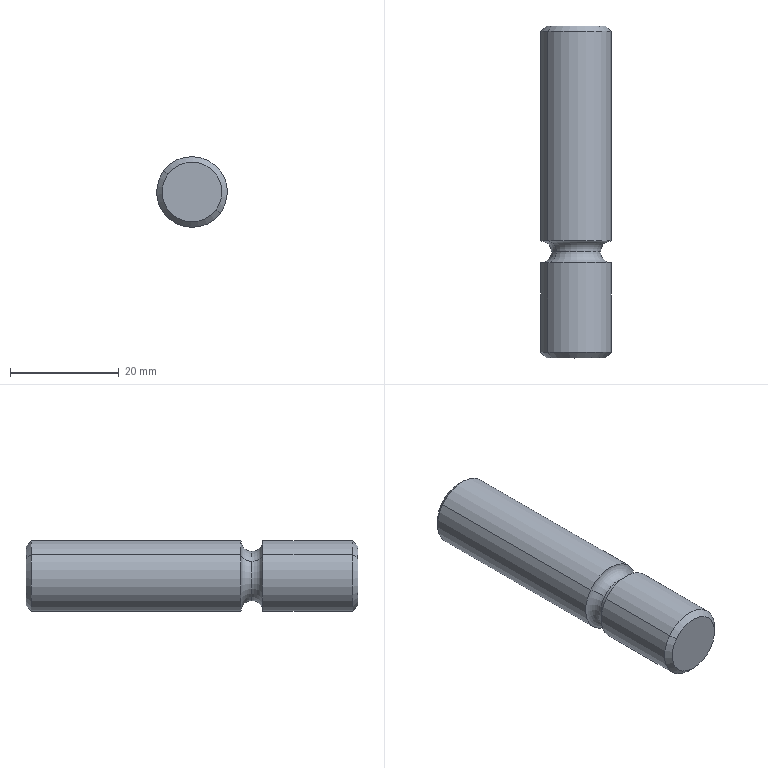Component | SolidWorks | 18-1 | 1 solid | 14 faces | box 13 x 61 x 13 mm | volume 7835 mm3 | torus 4 | cylinder 4 | cone 4 | plane 2 | commonest cylinder face diameters 13 x4
build123d program:
from build123d import *

# Parameters (mm, degrees)
SKETCH1_R           = 6.5
BOSS_EXTRUDE1_DEPTH = 61
CHAMFER1_SIZE       = 1
SKETCH2_R           = 2


with BuildPart() as part:
    # Sketch1 → Boss-Extrude1 (new body)
    with BuildSketch(Plane(origin=(0, 0, 0), x_dir=(0, 0, -1), z_dir=(1, 0, 0))):
        with Locations(Location((0, 0, 0), (0, 0, 180))):
            Circle(SKETCH1_R)
    extrude(amount=BOSS_EXTRUDE1_DEPTH)

    # Chamfer1
    chamfer1_edges = [part.edges().sort_by_distance(p)[0] for p in [
        (0, 0, -6.5),
        (61, 0, -6.5),
    ]]
    chamfer(chamfer1_edges, length=CHAMFER1_SIZE)

    # Sketch2 → Cut-Revolve1 (revolve, cut)
    with BuildSketch(Plane.XY, mode=Mode.PRIVATE) as cut_revolve1_sk:
        with Locations((19.5, 6.5)):
            Circle(SKETCH2_R)
    revolve(cut_revolve1_sk.sketch.rotate(Axis((0, 0, 0), (1, 0, 0)), 90), axis=Axis((0, 0, 0), (1, 0, 0)), mode=Mode.SUBTRACT)


solid = part.part

# Placed as in the assembly
solid = solid.moved(Location((-149.043, 247.491, 673.144), (0, 0, 90)))
STEP:
#1=COLOUR_RGB('',0.7922,0.8196,0.9333);
#2=FILL_AREA_STYLE_COLOUR('',#1);
#3=FILL_AREA_STYLE('',(#2));
#4=SURFACE_STYLE_FILL_AREA(#3);
#5=SURFACE_SIDE_STYLE('',(#4));
#6=SURFACE_STYLE_USAGE(.BOTH.,#5);
#7=PRESENTATION_STYLE_ASSIGNMENT((#6));
#8=CARTESIAN_POINT('',(-6.072,10.433,26.656));
#9=VERTEX_POINT('',#8);
#10=CARTESIAN_POINT('',(-6.009,10.511,26.609));
#11=VERTEX_POINT('',#10);
#12=CARTESIAN_POINT('',(-6.072,10.511,26.656));
#13=DIRECTION('',(0.6039,0.,0.797));
#14=DIRECTION('',(0.797,0.,-0.6039));
#15=AXIS2_PLACEMENT_3D('',#12,#13,#14);
#16=CIRCLE('',#15,0.07874);
#17=EDGE_CURVE('',#9,#11,#16,.T.);
#18=ORIENTED_EDGE('',*,*,#17,.T.);
#19=CARTESIAN_POINT('',(-5.727,10.511,26.395));
#20=VERTEX_POINT('',#19);
#21=CARTESIAN_POINT('',(-5.868,10.511,26.502));
#22=DIRECTION('',(0.,-1.,0.));
#23=DIRECTION('',(0.,0.,-1.));
#24=AXIS2_PLACEMENT_3D('',#21,#22,#23);
#25=CIRCLE('',#24,0.1772);
#26=EDGE_CURVE('',#11,#20,#25,.T.);
#27=ORIENTED_EDGE('',*,*,#26,.T.);
#28=CARTESIAN_POINT('',(-5.664,10.433,26.347));
#29=VERTEX_POINT('',#28);
#30=CARTESIAN_POINT('',(-5.664,10.511,26.347));
#31=DIRECTION('',(-0.6039,-0.,-0.797));
#32=DIRECTION('',(-0.797,0.,0.6039));
#33=AXIS2_PLACEMENT_3D('',#30,#31,#32);
#34=CIRCLE('',#33,0.07874);
#35=EDGE_CURVE('',#29,#20,#34,.T.);
#36=ORIENTED_EDGE('',*,*,#35,.F.);
#37=CARTESIAN_POINT('',(-5.868,10.433,26.502));
#38=DIRECTION('',(-0.,1.,-0.));
#39=DIRECTION('',(0.797,0.,-0.6039));
#40=AXIS2_PLACEMENT_3D('',#37,#38,#39);
#41=CIRCLE('',#40,0.2559);
#42=EDGE_CURVE('',#29,#9,#41,.T.);
#43=ORIENTED_EDGE('',*,*,#42,.T.);
#44=EDGE_LOOP('',(#18,#27,#36,#43));
#45=FACE_OUTER_BOUND('',#44,.T.);
#46=CARTESIAN_POINT('',(-5.868,10.511,26.502));
#47=DIRECTION('',(0.,-1.,0.));
#48=DIRECTION('',(-0.797,0.,0.6039));
#49=AXIS2_PLACEMENT_3D('',#46,#47,#48);
#50=TOROIDAL_SURFACE('',#49,0.2559,0.07874);
#51=ADVANCED_FACE('',(#45),#50,.F.);
#52=ORIENTED_EDGE('',*,*,#35,.T.);
#53=CARTESIAN_POINT('',(-5.868,10.511,26.502));
#54=DIRECTION('',(0.,-1.,0.));
#55=DIRECTION('',(0.,0.,-1.));
#56=AXIS2_PLACEMENT_3D('',#53,#54,#55);
#57=CIRCLE('',#56,0.1772);
#58=EDGE_CURVE('',#20,#11,#57,.T.);
#59=ORIENTED_EDGE('',*,*,#58,.T.);
#60=ORIENTED_EDGE('',*,*,#17,.F.);
#61=CARTESIAN_POINT('',(-5.868,10.433,26.502));
#62=DIRECTION('',(-0.,1.,-0.));
#63=DIRECTION('',(0.797,0.,-0.6039));
#64=AXIS2_PLACEMENT_3D('',#61,#62,#63);
#65=CIRCLE('',#64,0.2559);
#66=EDGE_CURVE('',#9,#29,#65,.T.);
#67=ORIENTED_EDGE('',*,*,#66,.T.);
#68=EDGE_LOOP('',(#52,#59,#60,#67));
#69=FACE_OUTER_BOUND('',#68,.T.);
#70=CARTESIAN_POINT('',(-5.868,10.511,26.502));
#71=DIRECTION('',(0.,-1.,0.));
#72=DIRECTION('',(-0.797,0.,0.6039));
#73=AXIS2_PLACEMENT_3D('',#70,#71,#72);
#74=TOROIDAL_SURFACE('',#73,0.2559,0.07874);
#75=ADVANCED_FACE('',(#69),#74,.F.);
#76=CARTESIAN_POINT('',(-6.072,12.106,26.656));
#77=VERTEX_POINT('',#76);
#78=CARTESIAN_POINT('',(-5.664,12.106,26.347));
#79=VERTEX_POINT('',#78);
#80=CARTESIAN_POINT('',(-5.868,12.106,26.502));
#81=DIRECTION('',(0.,-1.,0.));
#82=DIRECTION('',(0.797,0.,-0.6039));
#83=AXIS2_PLACEMENT_3D('',#80,#81,#82);
#84=CIRCLE('',#83,0.2559);
#85=EDGE_CURVE('',#77,#79,#84,.T.);
#86=ORIENTED_EDGE('',*,*,#85,.T.);
#87=CARTESIAN_POINT('',(-5.664,10.59,26.347));
#88=VERTEX_POINT('',#87);
#89=CARTESIAN_POINT('',(-5.664,12.145,26.347));
#90=DIRECTION('',(0.,-1.,0.));
#91=VECTOR('',#90,39.37);
#92=LINE('',#89,#91);
#93=EDGE_CURVE('',#79,#88,#92,.T.);
#94=ORIENTED_EDGE('',*,*,#93,.T.);
#95=CARTESIAN_POINT('',(-6.072,10.59,26.656));
#96=VERTEX_POINT('',#95);
#97=CARTESIAN_POINT('',(-5.868,10.59,26.502));
#98=DIRECTION('',(0.,-1.,0.));
#99=DIRECTION('',(-0.797,0.,0.6039));
#100=AXIS2_PLACEMENT_3D('',#97,#98,#99);
#101=CIRCLE('',#100,0.2559);
#102=EDGE_CURVE('',#96,#88,#101,.T.);
#103=ORIENTED_EDGE('',*,*,#102,.F.);
#104=CARTESIAN_POINT('',(-6.072,12.145,26.656));
#105=DIRECTION('',(0.,-1.,0.));
#106=VECTOR('',#105,39.37);
#107=LINE('',#104,#106);
#108=EDGE_CURVE('',#77,#96,#107,.T.);
#109=ORIENTED_EDGE('',*,*,#108,.F.);
#110=EDGE_LOOP('',(#86,#94,#103,#109));
#111=FACE_OUTER_BOUND('',#110,.T.);
#112=CARTESIAN_POINT('',(-5.868,12.145,26.502));
#113=DIRECTION('',(0.,-1.,0.));
#114=DIRECTION('',(-0.797,0.,0.6039));
#115=AXIS2_PLACEMENT_3D('',#112,#113,#114);
#116=CYLINDRICAL_SURFACE('',#115,0.2559);
#117=ADVANCED_FACE('',(#111),#116,.T.);
#118=CARTESIAN_POINT('',(-5.695,12.145,26.371));
#119=VERTEX_POINT('',#118);
#120=CARTESIAN_POINT('',(-6.04,12.145,26.632));
#121=VERTEX_POINT('',#120);
#122=CARTESIAN_POINT('',(-5.868,12.145,26.502));
#123=DIRECTION('',(-0.,1.,-0.));
#124=DIRECTION('',(0.797,0.,-0.6039));
#125=AXIS2_PLACEMENT_3D('',#122,#123,#124);
#126=CIRCLE('',#125,0.2165);
#127=EDGE_CURVE('',#119,#121,#126,.T.);
#128=ORIENTED_EDGE('',*,*,#127,.F.);
#129=CARTESIAN_POINT('',(-5.695,12.145,26.371));
#130=DIRECTION('',(0.5636,-0.7071,-0.427));
#131=VECTOR('',#130,39.37);
#132=LINE('',#129,#131);
#133=EDGE_CURVE('',#119,#79,#132,.T.);
#134=ORIENTED_EDGE('',*,*,#133,.T.);
#135=ORIENTED_EDGE('',*,*,#85,.F.);
#136=CARTESIAN_POINT('',(-6.04,12.145,26.632));
#137=DIRECTION('',(-0.5636,-0.7071,0.427));
#138=VECTOR('',#137,39.37);
#139=LINE('',#136,#138);
#140=EDGE_CURVE('',#121,#77,#139,.T.);
#141=ORIENTED_EDGE('',*,*,#140,.F.);
#142=EDGE_LOOP('',(#128,#134,#135,#141));
#143=FACE_OUTER_BOUND('',#142,.T.);
#144=CARTESIAN_POINT('',(-5.868,12.145,26.502));
#145=DIRECTION('',(0.,-1.,0.));
#146=DIRECTION('',(-0.797,0.,0.6039));
#147=AXIS2_PLACEMENT_3D('',#144,#145,#146);
#148=CONICAL_SURFACE('',#147,0.2165,0.7854);
#149=ADVANCED_FACE('',(#143),#148,.T.);
#150=ORIENTED_EDGE('',*,*,#58,.F.);
#151=CARTESIAN_POINT('',(-5.664,10.511,26.347));
#152=DIRECTION('',(-0.6039,-0.,-0.797));
#153=DIRECTION('',(-0.797,0.,0.6039));
#154=AXIS2_PLACEMENT_3D('',#151,#152,#153);
#155=CIRCLE('',#154,0.07874);
#156=EDGE_CURVE('',#20,#88,#155,.T.);
#157=ORIENTED_EDGE('',*,*,#156,.T.);
#158=CARTESIAN_POINT('',(-5.868,10.59,26.502));
#159=DIRECTION('',(0.,-1.,0.));
#160=DIRECTION('',(-0.797,0.,0.6039));
#161=AXIS2_PLACEMENT_3D('',#158,#159,#160);
#162=CIRCLE('',#161,0.2559);
#163=EDGE_CURVE('',#88,#96,#162,.T.);
#164=ORIENTED_EDGE('',*,*,#163,.T.);
#165=CARTESIAN_POINT('',(-6.072,10.511,26.656));
#166=DIRECTION('',(0.6039,0.,0.797));
#167=DIRECTION('',(0.797,0.,-0.6039));
#168=AXIS2_PLACEMENT_3D('',#165,#166,#167);
#169=CIRCLE('',#168,0.07874);
#170=EDGE_CURVE('',#11,#96,#169,.T.);
#171=ORIENTED_EDGE('',*,*,#170,.F.);
#172=EDGE_LOOP('',(#150,#157,#164,#171));
#173=FACE_OUTER_BOUND('',#172,.T.);
#174=CARTESIAN_POINT('',(-5.868,10.511,26.502));
#175=DIRECTION('',(0.,-1.,0.));
#176=DIRECTION('',(-0.797,0.,0.6039));
#177=AXIS2_PLACEMENT_3D('',#174,#175,#176);
#178=TOROIDAL_SURFACE('',#177,0.2559,0.07874);
#179=ADVANCED_FACE('',(#173),#178,.F.);
#180=CARTESIAN_POINT('',(-6.04,9.744,26.632));
#181=VERTEX_POINT('',#180);
#182=CARTESIAN_POINT('',(-5.695,9.744,26.371));
#183=VERTEX_POINT('',#182);
#184=CARTESIAN_POINT('',(-5.868,9.744,26.502));
#185=DIRECTION('',(0.,-1.,0.));
#186=DIRECTION('',(0.797,0.,-0.6039));
#187=AXIS2_PLACEMENT_3D('',#184,#185,#186);
#188=CIRCLE('',#187,0.2165);
#189=EDGE_CURVE('',#181,#183,#188,.T.);
#190=ORIENTED_EDGE('',*,*,#189,.F.);
#191=CARTESIAN_POINT('',(-6.072,9.783,26.656));
#192=VERTEX_POINT('',#191);
#193=CARTESIAN_POINT('',(-6.072,9.783,26.656));
#194=DIRECTION('',(-0.5636,0.7071,0.427));
#195=VECTOR('',#194,39.37);
#196=LINE('',#193,#195);
#197=EDGE_CURVE('',#181,#192,#196,.T.);
#198=ORIENTED_EDGE('',*,*,#197,.T.);
#199=CARTESIAN_POINT('',(-5.664,9.783,26.347));
#200=VERTEX_POINT('',#199);
#201=CARTESIAN_POINT('',(-5.868,9.783,26.502));
#202=DIRECTION('',(-0.,1.,-0.));
#203=DIRECTION('',(0.797,0.,-0.6039));
#204=AXIS2_PLACEMENT_3D('',#201,#202,#203);
#205=CIRCLE('',#204,0.2559);
#206=EDGE_CURVE('',#200,#192,#205,.T.);
#207=ORIENTED_EDGE('',*,*,#206,.F.);
#208=CARTESIAN_POINT('',(-5.664,9.783,26.347));
#209=DIRECTION('',(0.5636,0.7071,-0.427));
#210=VECTOR('',#209,39.37);
#211=LINE('',#208,#210);
#212=EDGE_CURVE('',#183,#200,#211,.T.);
#213=ORIENTED_EDGE('',*,*,#212,.F.);
#214=EDGE_LOOP('',(#190,#198,#207,#213));
#215=FACE_OUTER_BOUND('',#214,.T.);
#216=CARTESIAN_POINT('',(-5.868,9.783,26.502));
#217=DIRECTION('',(-0.,1.,-0.));
#218=DIRECTION('',(0.797,0.,-0.6039));
#219=AXIS2_PLACEMENT_3D('',#216,#217,#218);
#220=CONICAL_SURFACE('',#219,0.2559,0.7854);
#221=ADVANCED_FACE('',(#215),#220,.T.);
#222=ORIENTED_EDGE('',*,*,#42,.F.);
#223=CARTESIAN_POINT('',(-5.664,12.145,26.347));
#224=DIRECTION('',(0.,-1.,0.));
#225=VECTOR('',#224,39.37);
#226=LINE('',#223,#225);
#227=EDGE_CURVE('',#29,#200,#226,.T.);
#228=ORIENTED_EDGE('',*,*,#227,.T.);
#229=ORIENTED_EDGE('',*,*,#206,.T.);
#230=CARTESIAN_POINT('',(-6.072,12.145,26.656));
#231=DIRECTION('',(0.,-1.,0.));
#232=VECTOR('',#231,39.37);
#233=LINE('',#230,#232);
#234=EDGE_CURVE('',#9,#192,#233,.T.);
#235=ORIENTED_EDGE('',*,*,#234,.F.);
#236=EDGE_LOOP('',(#222,#228,#229,#235));
#237=FACE_OUTER_BOUND('',#236,.T.);
#238=CARTESIAN_POINT('',(-5.868,12.145,26.502));
#239=DIRECTION('',(0.,-1.,0.));
#240=DIRECTION('',(-0.797,0.,0.6039));
#241=AXIS2_PLACEMENT_3D('',#238,#239,#240);
#242=CYLINDRICAL_SURFACE('',#241,0.2559);
#243=ADVANCED_FACE('',(#237),#242,.T.);
#244=ORIENTED_EDGE('',*,*,#227,.F.);
#245=ORIENTED_EDGE('',*,*,#66,.F.);
#246=ORIENTED_EDGE('',*,*,#234,.T.);
#247=CARTESIAN_POINT('',(-5.868,9.783,26.502));
#248=DIRECTION('',(-0.,1.,-0.));
#249=DIRECTION('',(0.797,0.,-0.6039));
#250=AXIS2_PLACEMENT_3D('',#247,#248,#249);
#251=CIRCLE('',#250,0.2559);
#252=EDGE_CURVE('',#192,#200,#251,.T.);
#253=ORIENTED_EDGE('',*,*,#252,.T.);
#254=EDGE_LOOP('',(#244,#245,#246,#253));
#255=FACE_OUTER_BOUND('',#254,.T.);
#256=CARTESIAN_POINT('',(-5.868,12.145,26.502));
#257=DIRECTION('',(0.,-1.,0.));
#258=DIRECTION('',(-0.797,0.,0.6039));
#259=AXIS2_PLACEMENT_3D('',#256,#257,#258);
#260=CYLINDRICAL_SURFACE('',#259,0.2559);
#261=ADVANCED_FACE('',(#255),#260,.T.);
#262=CARTESIAN_POINT('',(-5.868,9.744,26.502));
#263=DIRECTION('',(0.,-1.,0.));
#264=DIRECTION('',(0.797,0.,-0.6039));
#265=AXIS2_PLACEMENT_3D('',#262,#263,#264);
#266=CIRCLE('',#265,0.2165);
#267=EDGE_CURVE('',#183,#181,#266,.T.);
#268=ORIENTED_EDGE('',*,*,#267,.T.);
#269=ORIENTED_EDGE('',*,*,#189,.T.);
#270=EDGE_LOOP('',(#268,#269));
#271=FACE_OUTER_BOUND('',#270,.T.);
#272=CARTESIAN_POINT('',(-5.868,9.744,26.502));
#273=DIRECTION('',(-0.,1.,-0.));
#274=DIRECTION('',(0.797,-0.,-0.6039));
#275=AXIS2_PLACEMENT_3D('',#272,#273,#274);
#276=PLANE('',#275);
#277=ADVANCED_FACE('',(#271),#276,.F.);
#278=ORIENTED_EDGE('',*,*,#197,.F.);
#279=ORIENTED_EDGE('',*,*,#267,.F.);
#280=ORIENTED_EDGE('',*,*,#212,.T.);
#281=ORIENTED_EDGE('',*,*,#252,.F.);
#282=EDGE_LOOP('',(#278,#279,#280,#281));
#283=FACE_OUTER_BOUND('',#282,.T.);
#284=CARTESIAN_POINT('',(-5.868,9.783,26.502));
#285=DIRECTION('',(-0.,1.,-0.));
#286=DIRECTION('',(0.797,0.,-0.6039));
#287=AXIS2_PLACEMENT_3D('',#284,#285,#286);
#288=CONICAL_SURFACE('',#287,0.2559,0.7854);
#289=ADVANCED_FACE('',(#283),#288,.T.);
#290=ORIENTED_EDGE('',*,*,#26,.F.);
#291=ORIENTED_EDGE('',*,*,#170,.T.);
#292=ORIENTED_EDGE('',*,*,#102,.T.);
#293=ORIENTED_EDGE('',*,*,#156,.F.);
#294=EDGE_LOOP('',(#290,#291,#292,#293));
#295=FACE_OUTER_BOUND('',#294,.T.);
#296=CARTESIAN_POINT('',(-5.868,10.511,26.502));
#297=DIRECTION('',(0.,-1.,0.));
#298=DIRECTION('',(-0.797,0.,0.6039));
#299=AXIS2_PLACEMENT_3D('',#296,#297,#298);
#300=TOROIDAL_SURFACE('',#299,0.2559,0.07874);
#301=ADVANCED_FACE('',(#295),#300,.F.);
#302=CARTESIAN_POINT('',(-5.868,12.145,26.502));
#303=DIRECTION('',(-0.,1.,-0.));
#304=DIRECTION('',(0.797,0.,-0.6039));
#305=AXIS2_PLACEMENT_3D('',#302,#303,#304);
#306=CIRCLE('',#305,0.2165);
#307=EDGE_CURVE('',#121,#119,#306,.T.);
#308=ORIENTED_EDGE('',*,*,#307,.T.);
#309=ORIENTED_EDGE('',*,*,#127,.T.);
#310=EDGE_LOOP('',(#308,#309));
#311=FACE_OUTER_BOUND('',#310,.T.);
#312=CARTESIAN_POINT('',(-5.868,12.145,26.502));
#313=DIRECTION('',(-0.,1.,-0.));
#314=DIRECTION('',(0.797,-0.,-0.6039));
#315=AXIS2_PLACEMENT_3D('',#312,#313,#314);
#316=PLANE('',#315);
#317=ADVANCED_FACE('',(#311),#316,.T.);
#318=ORIENTED_EDGE('',*,*,#133,.F.);
#319=ORIENTED_EDGE('',*,*,#307,.F.);
#320=ORIENTED_EDGE('',*,*,#140,.T.);
#321=CARTESIAN_POINT('',(-5.868,12.106,26.502));
#322=DIRECTION('',(0.,-1.,0.));
#323=DIRECTION('',(0.797,0.,-0.6039));
#324=AXIS2_PLACEMENT_3D('',#321,#322,#323);
#325=CIRCLE('',#324,0.2559);
#326=EDGE_CURVE('',#79,#77,#325,.T.);
#327=ORIENTED_EDGE('',*,*,#326,.F.);
#328=EDGE_LOOP('',(#318,#319,#320,#327));
#329=FACE_OUTER_BOUND('',#328,.T.);
#330=CARTESIAN_POINT('',(-5.868,12.145,26.502));
#331=DIRECTION('',(0.,-1.,0.));
#332=DIRECTION('',(-0.797,0.,0.6039));
#333=AXIS2_PLACEMENT_3D('',#330,#331,#332);
#334=CONICAL_SURFACE('',#333,0.2165,0.7854);
#335=ADVANCED_FACE('',(#329),#334,.T.);
#336=ORIENTED_EDGE('',*,*,#93,.F.);
#337=ORIENTED_EDGE('',*,*,#326,.T.);
#338=ORIENTED_EDGE('',*,*,#108,.T.);
#339=ORIENTED_EDGE('',*,*,#163,.F.);
#340=EDGE_LOOP('',(#336,#337,#338,#339));
#341=FACE_OUTER_BOUND('',#340,.T.);
#342=CARTESIAN_POINT('',(-5.868,12.145,26.502));
#343=DIRECTION('',(0.,-1.,0.));
#344=DIRECTION('',(-0.797,0.,0.6039));
#345=AXIS2_PLACEMENT_3D('',#342,#343,#344);
#346=CYLINDRICAL_SURFACE('',#345,0.2559);
#347=ADVANCED_FACE('',(#341),#346,.T.);
#348=CLOSED_SHELL('',(#51,#75,#117,#149,#179,#221,#243,#261,#277,#289,#301,#317,#335,#347));
#349=MANIFOLD_SOLID_BREP('',#348);
#350=STYLED_ITEM('',(#7),#349);
#351=PRESENTATION_LAYER_ASSIGNMENT('','',(#350));
#352=CARTESIAN_POINT('',(0.,0.,0.));
#353=DIRECTION('',(0.,0.,1.));
#354=DIRECTION('',(1.,0.,0.));
#355=AXIS2_PLACEMENT_3D('',#352,#353,#354);
#356=(LENGTH_UNIT()NAMED_UNIT(*)SI_UNIT($,.METRE.));
#357=LENGTH_MEASURE_WITH_UNIT(LENGTH_MEASURE(0.0254),#356);
#358=DIMENSIONAL_EXPONENTS(1.,0.,0.,0.,0.,0.,0.);
#359=(CONVERSION_BASED_UNIT('',#357)LENGTH_UNIT()NAMED_UNIT(#358));
#360=UNCERTAINTY_MEASURE_WITH_UNIT(LENGTH_MEASURE(0.00001),#359,'','');
#361=(NAMED_UNIT(*)PLANE_ANGLE_UNIT()SI_UNIT($,.RADIAN.));
#362=(NAMED_UNIT(*)SI_UNIT($,.STERADIAN.)SOLID_ANGLE_UNIT());
#363=(GEOMETRIC_REPRESENTATION_CONTEXT(3)GLOBAL_UNCERTAINTY_ASSIGNED_CONTEXT((#360))GLOBAL_UNIT_ASSIGNED_CONTEXT((#359,#361,#362))REPRESENTATION_CONTEXT('',''));
#364=ADVANCED_BREP_SHAPE_REPRESENTATION('',(#349,#355),#363);
#365=(LENGTH_UNIT()NAMED_UNIT(*)SI_UNIT($,.METRE.));
#366=LENGTH_MEASURE_WITH_UNIT(LENGTH_MEASURE(0.0254),#365);
#367=DIMENSIONAL_EXPONENTS(1.,0.,0.,0.,0.,0.,0.);
#368=(CONVERSION_BASED_UNIT('',#366)LENGTH_UNIT()NAMED_UNIT(#367));
#369=UNCERTAINTY_MEASURE_WITH_UNIT(LENGTH_MEASURE(0.00001),#368,'','');
#370=(NAMED_UNIT(*)PLANE_ANGLE_UNIT()SI_UNIT($,.RADIAN.));
#371=(NAMED_UNIT(*)SI_UNIT($,.STERADIAN.)SOLID_ANGLE_UNIT());
#372=(GEOMETRIC_REPRESENTATION_CONTEXT(3)GLOBAL_UNCERTAINTY_ASSIGNED_CONTEXT((#369))GLOBAL_UNIT_ASSIGNED_CONTEXT((#368,#370,#371))REPRESENTATION_CONTEXT('',''));
#373=MECHANICAL_DESIGN_GEOMETRIC_PRESENTATION_REPRESENTATION('',(#350),#372);